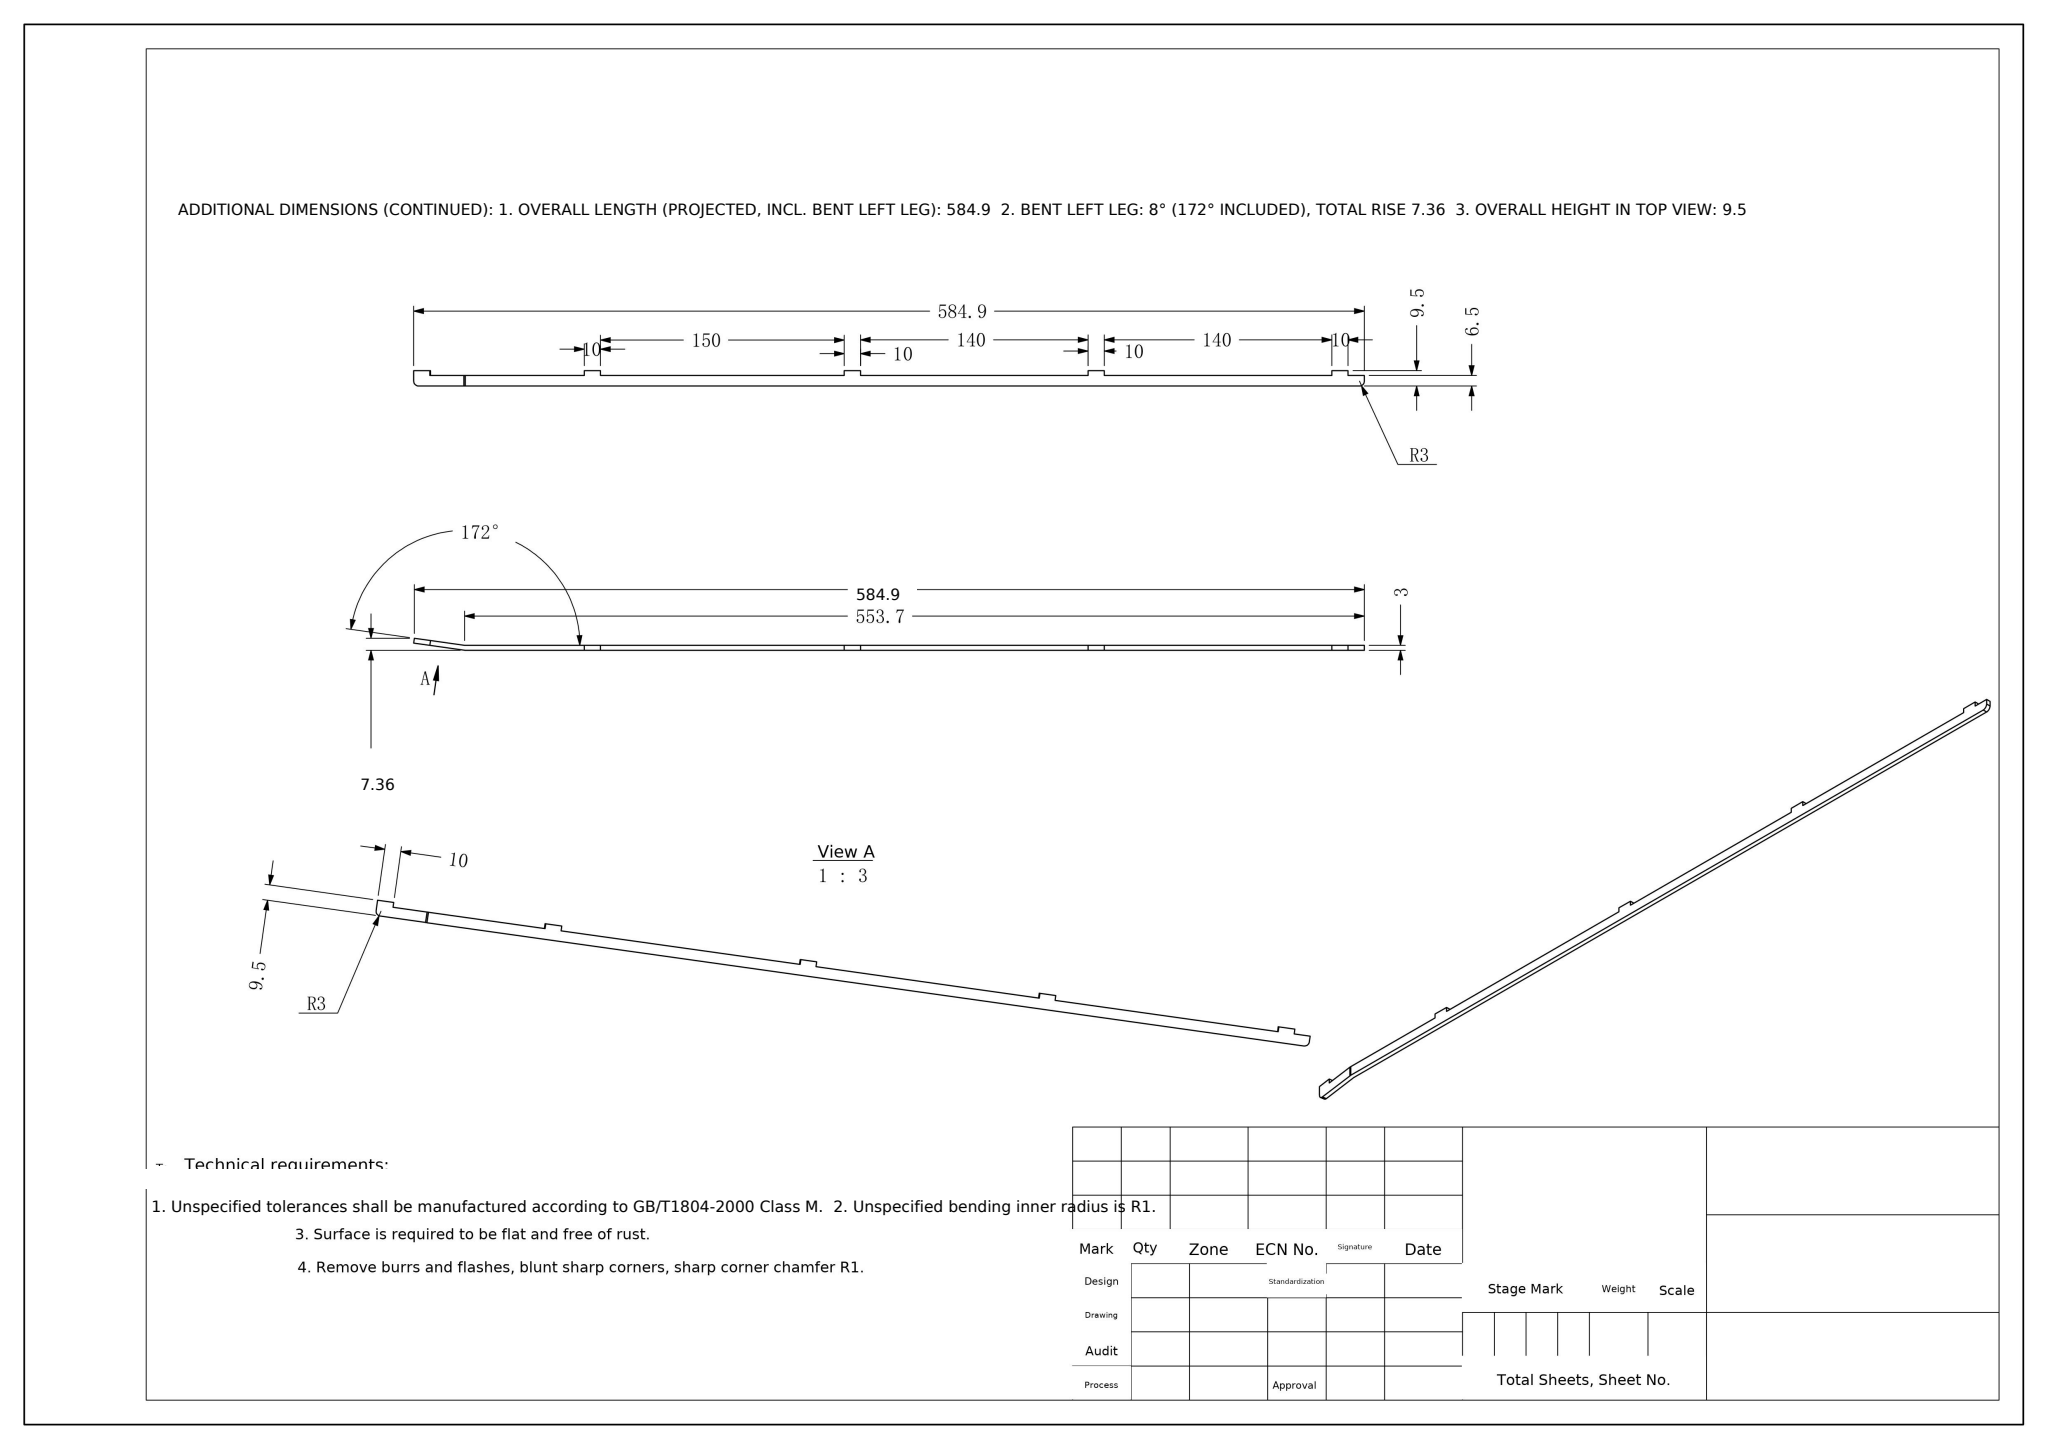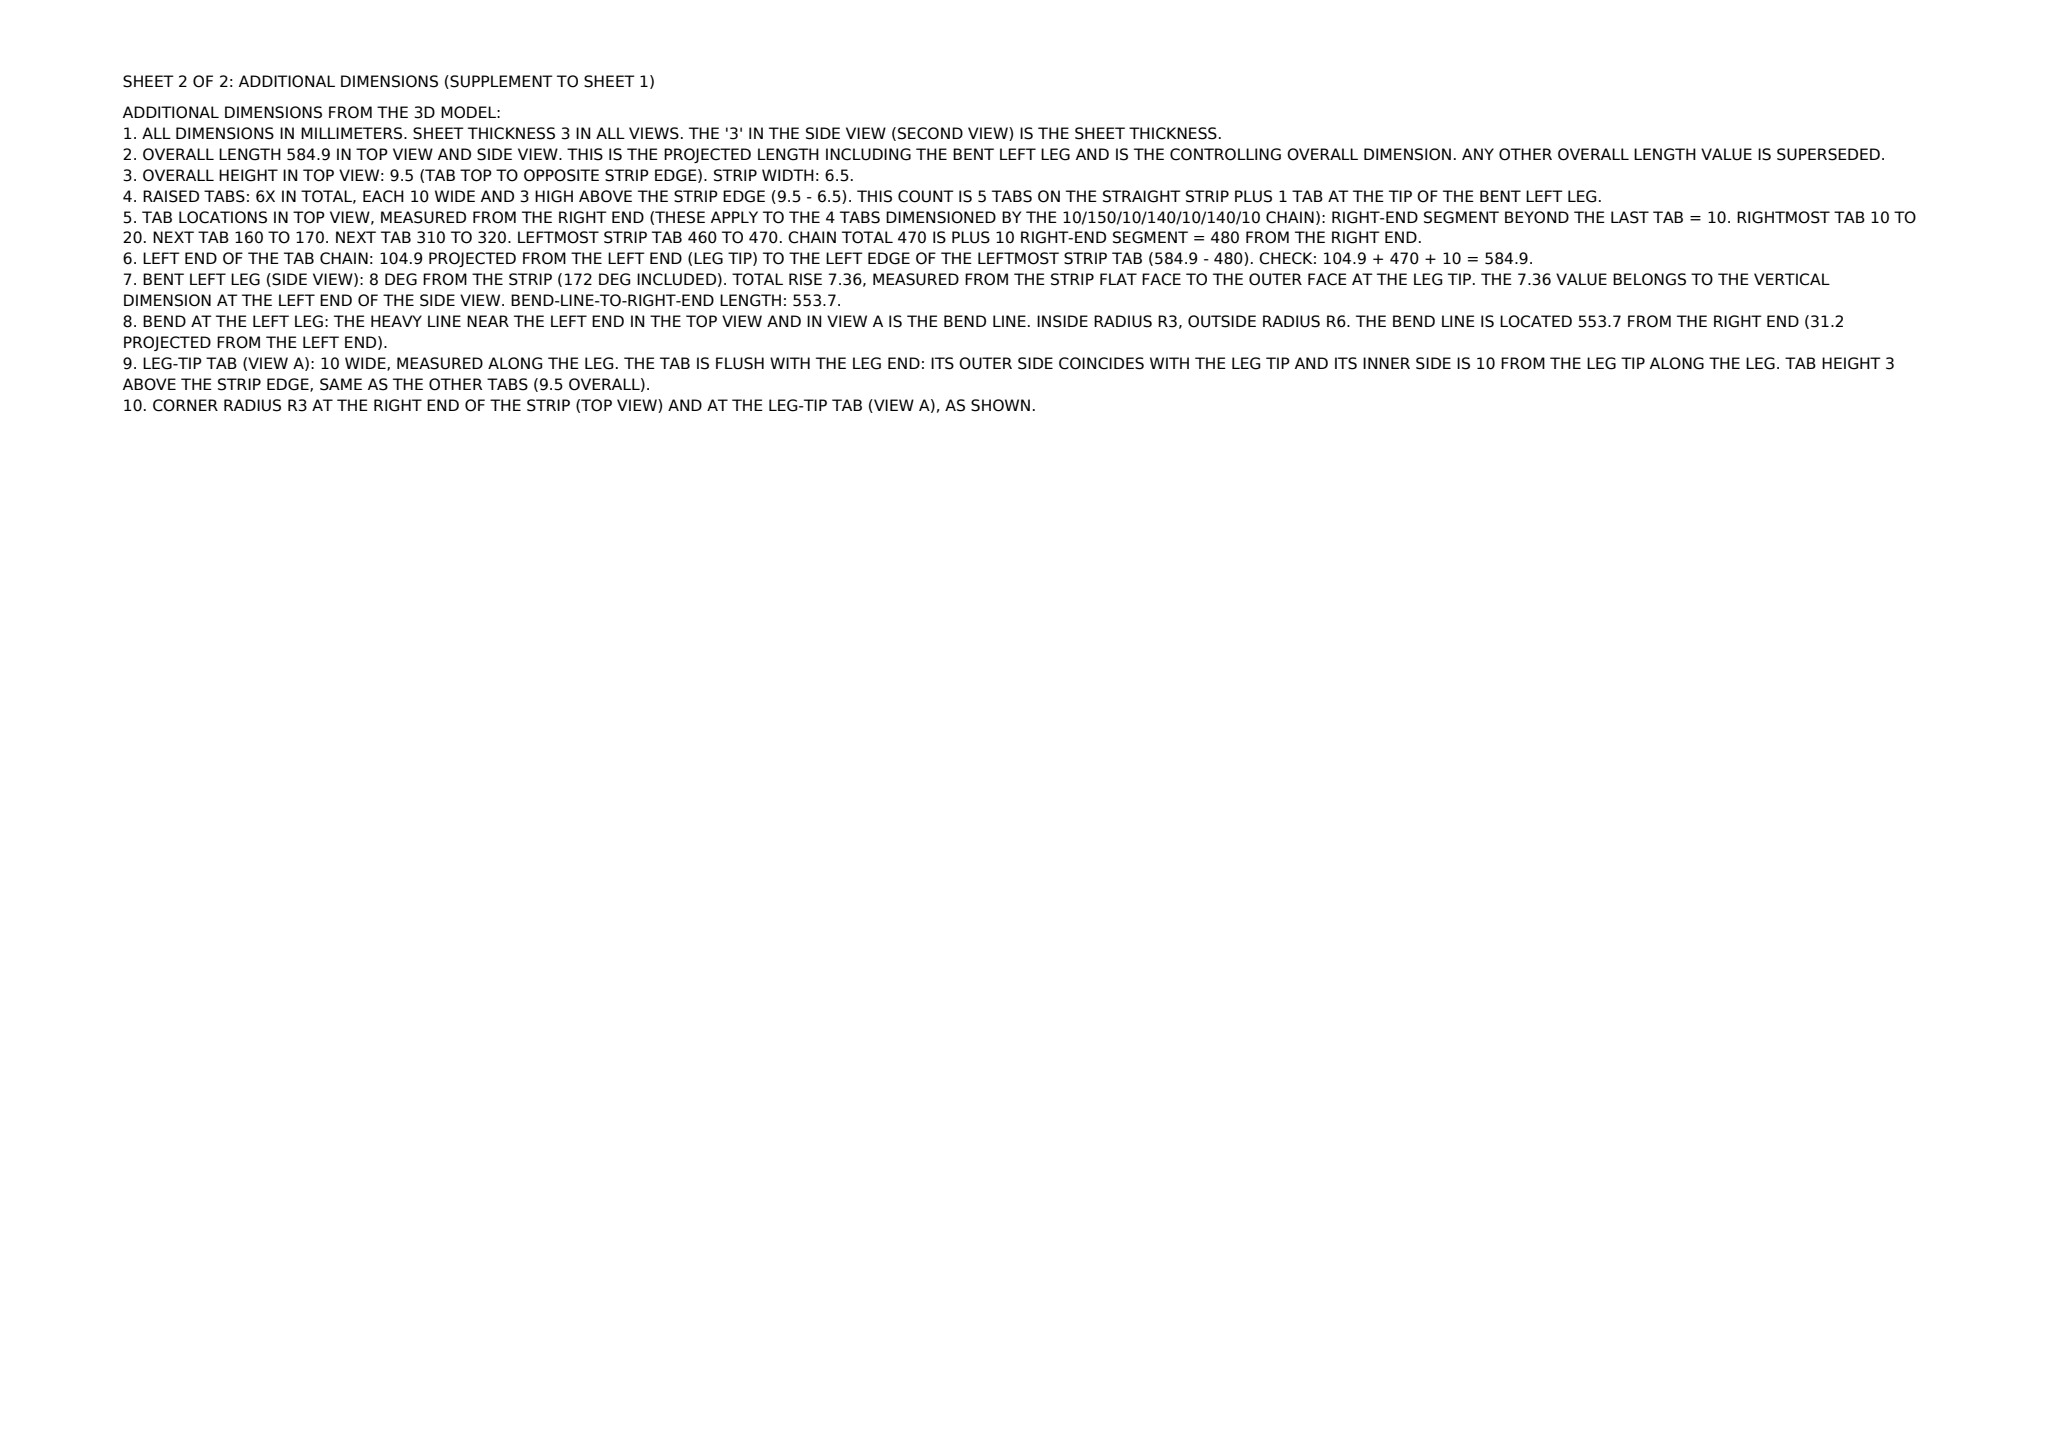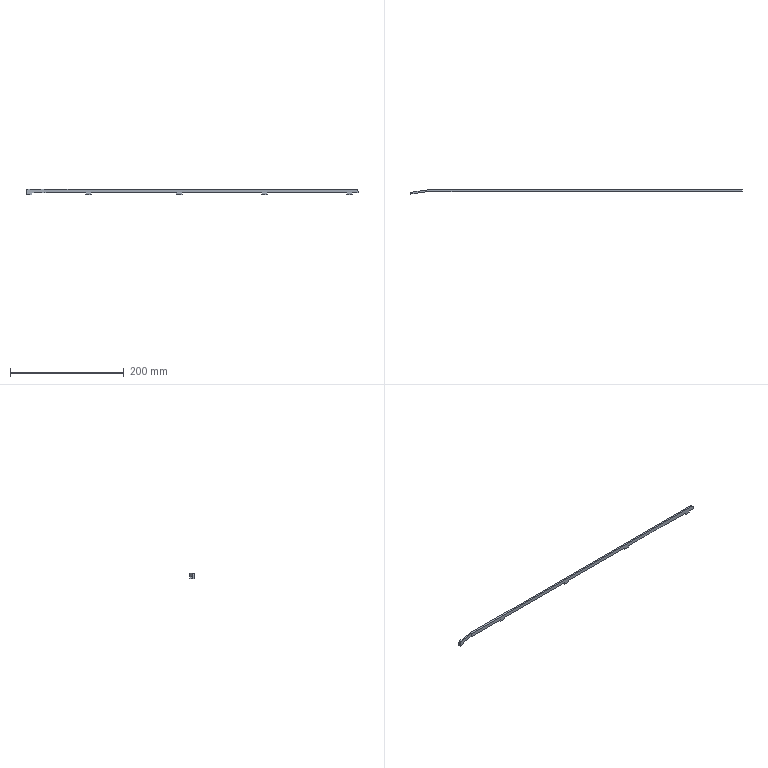Part | NX | mm | 1 solid | 30 faces | box 584.9 x 7.36 x 9.5 mm | volume 11846 mm3 | plane 26 | cylinder 4 | commonest cylinder face diameters 6 x3 12 x1